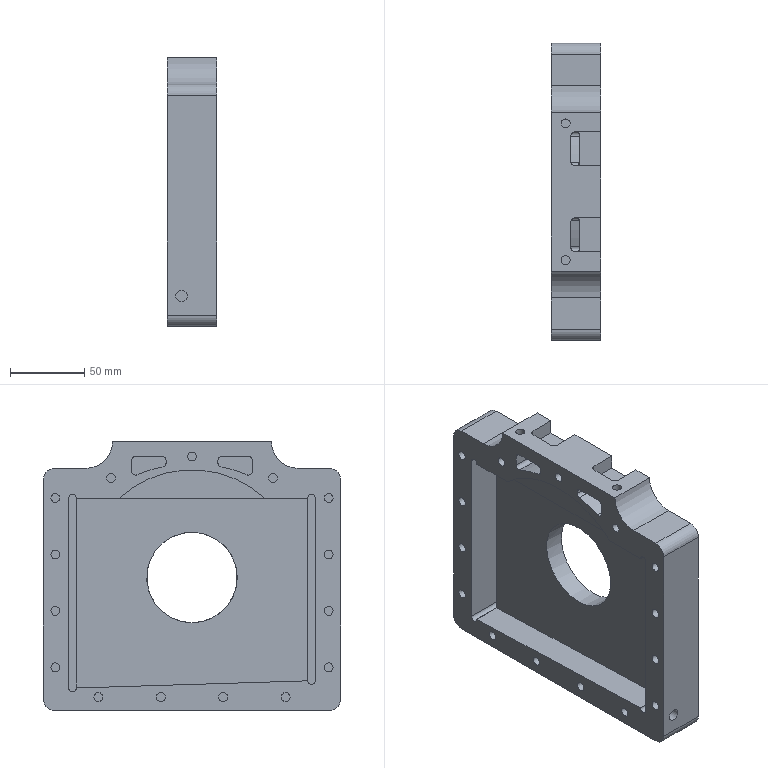Component | NX | CYLINDER_BODY | 1 solid | 126 faces | volume 662370 mm3 | plane 65 | cylinder 61 | commonest cylinder face diameters 6 x33 5 x16 15 x4 36 x2 194 x2 8 x2 61 x1 145 x1